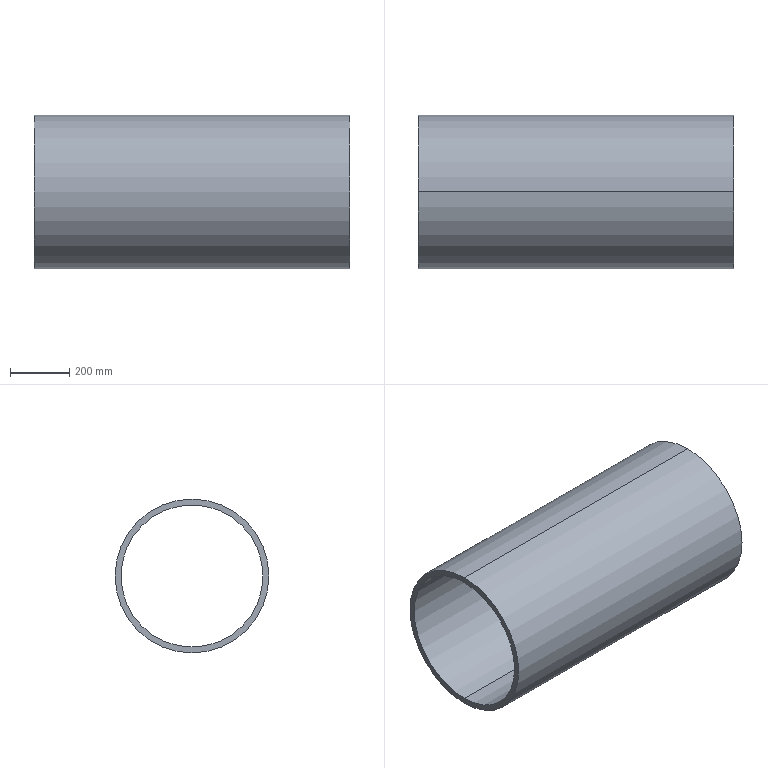Component | SolidWorks | Cev-osnovna-1 | 1 solid | 6 faces | box 1070 x 521 x 521 mm | volume 33682271 mm3 | cylinder 4 | plane 2 | commonest cylinder face diameters 481 x2 521 x2
build123d program:
from build123d import *

# Parameters (mm, degrees)
BOSS_EXTRUDE1_DEPTH      = 70
BOSS_EXTRUDE1_DEPTH_BACK = 1000
SKETCH1_R                = 260.5
SKETCH1_R_2              = 240.5


with BuildPart() as part:
    # Sketch1 → Boss-Extrude1 (new, two sides: drawn at the far end of the back side and taken through both)
    with BuildSketch(Plane.XY.offset(-7660).offset(-BOSS_EXTRUDE1_DEPTH_BACK)):
        Circle(SKETCH1_R)
        Circle(SKETCH1_R_2, mode=Mode.SUBTRACT)
    extrude(amount=BOSS_EXTRUDE1_DEPTH + BOSS_EXTRUDE1_DEPTH_BACK)


solid = part.part

# Placed as in the assembly
solid = solid.moved(Location((7660, 0, 0), (0, 90, 0)))
STEP:
#1=COLOUR_RGB('',0.7922,0.8196,0.9333);
#2=FILL_AREA_STYLE_COLOUR('',#1);
#3=FILL_AREA_STYLE('',(#2));
#4=SURFACE_STYLE_FILL_AREA(#3);
#5=SURFACE_SIDE_STYLE('',(#4));
#6=SURFACE_STYLE_USAGE(.BOTH.,#5);
#7=PRESENTATION_STYLE_ASSIGNMENT((#6));
#8=CARTESIAN_POINT('',(-39.37,0.,9.469));
#9=VERTEX_POINT('',#8);
#10=CARTESIAN_POINT('',(-39.37,0.,-9.469));
#11=VERTEX_POINT('',#10);
#12=CARTESIAN_POINT('',(-39.37,0.,-0.));
#13=DIRECTION('',(1.,0.,0.));
#14=DIRECTION('',(0.,0.,-1.));
#15=AXIS2_PLACEMENT_3D('',#12,#13,#14);
#16=CIRCLE('',#15,9.469);
#17=EDGE_CURVE('',#9,#11,#16,.T.);
#18=ORIENTED_EDGE('',*,*,#17,.F.);
#19=CARTESIAN_POINT('',(2.756,0.,9.469));
#20=VERTEX_POINT('',#19);
#21=CARTESIAN_POINT('',(-39.37,0.,9.469));
#22=DIRECTION('',(1.,0.,0.));
#23=VECTOR('',#22,39.37);
#24=LINE('',#21,#23);
#25=EDGE_CURVE('',#9,#20,#24,.T.);
#26=ORIENTED_EDGE('',*,*,#25,.T.);
#27=CARTESIAN_POINT('',(2.756,0.,-9.469));
#28=VERTEX_POINT('',#27);
#29=CARTESIAN_POINT('',(2.756,0.,0.));
#30=DIRECTION('',(1.,0.,0.));
#31=DIRECTION('',(0.,0.,-1.));
#32=AXIS2_PLACEMENT_3D('',#29,#30,#31);
#33=CIRCLE('',#32,9.469);
#34=EDGE_CURVE('',#20,#28,#33,.T.);
#35=ORIENTED_EDGE('',*,*,#34,.T.);
#36=CARTESIAN_POINT('',(-39.37,0.,-9.469));
#37=DIRECTION('',(1.,0.,0.));
#38=VECTOR('',#37,39.37);
#39=LINE('',#36,#38);
#40=EDGE_CURVE('',#11,#28,#39,.T.);
#41=ORIENTED_EDGE('',*,*,#40,.F.);
#42=EDGE_LOOP('',(#18,#26,#35,#41));
#43=FACE_OUTER_BOUND('',#42,.T.);
#44=CARTESIAN_POINT('',(-39.37,0.,-0.));
#45=DIRECTION('',(1.,0.,0.));
#46=DIRECTION('',(0.,0.,-1.));
#47=AXIS2_PLACEMENT_3D('',#44,#45,#46);
#48=CYLINDRICAL_SURFACE('',#47,9.469);
#49=ADVANCED_FACE('',(#43),#48,.F.);
#50=CARTESIAN_POINT('',(-39.37,0.,-10.256));
#51=VERTEX_POINT('',#50);
#52=CARTESIAN_POINT('',(-39.37,0.,10.256));
#53=VERTEX_POINT('',#52);
#54=CARTESIAN_POINT('',(-39.37,0.,-0.));
#55=DIRECTION('',(1.,0.,0.));
#56=DIRECTION('',(0.,0.,-1.));
#57=AXIS2_PLACEMENT_3D('',#54,#55,#56);
#58=CIRCLE('',#57,10.256);
#59=EDGE_CURVE('',#51,#53,#58,.T.);
#60=ORIENTED_EDGE('',*,*,#59,.T.);
#61=CARTESIAN_POINT('',(2.756,0.,10.256));
#62=VERTEX_POINT('',#61);
#63=CARTESIAN_POINT('',(-39.37,0.,10.256));
#64=DIRECTION('',(1.,0.,0.));
#65=VECTOR('',#64,39.37);
#66=LINE('',#63,#65);
#67=EDGE_CURVE('',#53,#62,#66,.T.);
#68=ORIENTED_EDGE('',*,*,#67,.T.);
#69=CARTESIAN_POINT('',(2.756,0.,-10.256));
#70=VERTEX_POINT('',#69);
#71=CARTESIAN_POINT('',(2.756,0.,0.));
#72=DIRECTION('',(1.,0.,0.));
#73=DIRECTION('',(0.,0.,-1.));
#74=AXIS2_PLACEMENT_3D('',#71,#72,#73);
#75=CIRCLE('',#74,10.256);
#76=EDGE_CURVE('',#70,#62,#75,.T.);
#77=ORIENTED_EDGE('',*,*,#76,.F.);
#78=CARTESIAN_POINT('',(-39.37,0.,-10.256));
#79=DIRECTION('',(1.,0.,0.));
#80=VECTOR('',#79,39.37);
#81=LINE('',#78,#80);
#82=EDGE_CURVE('',#51,#70,#81,.T.);
#83=ORIENTED_EDGE('',*,*,#82,.F.);
#84=EDGE_LOOP('',(#60,#68,#77,#83));
#85=FACE_OUTER_BOUND('',#84,.T.);
#86=CARTESIAN_POINT('',(-39.37,0.,-0.));
#87=DIRECTION('',(1.,0.,0.));
#88=DIRECTION('',(0.,0.,-1.));
#89=AXIS2_PLACEMENT_3D('',#86,#87,#88);
#90=CYLINDRICAL_SURFACE('',#89,10.256);
#91=ADVANCED_FACE('',(#85),#90,.T.);
#92=ORIENTED_EDGE('',*,*,#67,.F.);
#93=CARTESIAN_POINT('',(-39.37,0.,-0.));
#94=DIRECTION('',(1.,0.,0.));
#95=DIRECTION('',(0.,0.,-1.));
#96=AXIS2_PLACEMENT_3D('',#93,#94,#95);
#97=CIRCLE('',#96,10.256);
#98=EDGE_CURVE('',#53,#51,#97,.T.);
#99=ORIENTED_EDGE('',*,*,#98,.T.);
#100=ORIENTED_EDGE('',*,*,#82,.T.);
#101=CARTESIAN_POINT('',(2.756,0.,0.));
#102=DIRECTION('',(1.,0.,0.));
#103=DIRECTION('',(0.,0.,-1.));
#104=AXIS2_PLACEMENT_3D('',#101,#102,#103);
#105=CIRCLE('',#104,10.256);
#106=EDGE_CURVE('',#62,#70,#105,.T.);
#107=ORIENTED_EDGE('',*,*,#106,.F.);
#108=EDGE_LOOP('',(#92,#99,#100,#107));
#109=FACE_OUTER_BOUND('',#108,.T.);
#110=CARTESIAN_POINT('',(-39.37,0.,-0.));
#111=DIRECTION('',(1.,0.,0.));
#112=DIRECTION('',(0.,0.,-1.));
#113=AXIS2_PLACEMENT_3D('',#110,#111,#112);
#114=CYLINDRICAL_SURFACE('',#113,10.256);
#115=ADVANCED_FACE('',(#109),#114,.T.);
#116=CARTESIAN_POINT('',(-39.37,0.,-0.));
#117=DIRECTION('',(1.,0.,0.));
#118=DIRECTION('',(0.,0.,-1.));
#119=AXIS2_PLACEMENT_3D('',#116,#117,#118);
#120=CIRCLE('',#119,9.469);
#121=EDGE_CURVE('',#11,#9,#120,.T.);
#122=ORIENTED_EDGE('',*,*,#121,.T.);
#123=ORIENTED_EDGE('',*,*,#17,.T.);
#124=EDGE_LOOP('',(#122,#123));
#125=FACE_BOUND('',#124,.T.);
#126=ORIENTED_EDGE('',*,*,#59,.F.);
#127=ORIENTED_EDGE('',*,*,#98,.F.);
#128=EDGE_LOOP('',(#126,#127));
#129=FACE_OUTER_BOUND('',#128,.T.);
#130=CARTESIAN_POINT('',(-39.37,0.,-0.));
#131=DIRECTION('',(1.,0.,0.));
#132=DIRECTION('',(0.,0.,-1.));
#133=AXIS2_PLACEMENT_3D('',#130,#131,#132);
#134=PLANE('',#133);
#135=ADVANCED_FACE('',(#125,#129),#134,.F.);
#136=ORIENTED_EDGE('',*,*,#25,.F.);
#137=ORIENTED_EDGE('',*,*,#121,.F.);
#138=ORIENTED_EDGE('',*,*,#40,.T.);
#139=CARTESIAN_POINT('',(2.756,0.,0.));
#140=DIRECTION('',(1.,0.,0.));
#141=DIRECTION('',(0.,0.,-1.));
#142=AXIS2_PLACEMENT_3D('',#139,#140,#141);
#143=CIRCLE('',#142,9.469);
#144=EDGE_CURVE('',#28,#20,#143,.T.);
#145=ORIENTED_EDGE('',*,*,#144,.T.);
#146=EDGE_LOOP('',(#136,#137,#138,#145));
#147=FACE_OUTER_BOUND('',#146,.T.);
#148=CARTESIAN_POINT('',(-39.37,0.,-0.));
#149=DIRECTION('',(1.,0.,0.));
#150=DIRECTION('',(0.,0.,-1.));
#151=AXIS2_PLACEMENT_3D('',#148,#149,#150);
#152=CYLINDRICAL_SURFACE('',#151,9.469);
#153=ADVANCED_FACE('',(#147),#152,.F.);
#154=ORIENTED_EDGE('',*,*,#76,.T.);
#155=ORIENTED_EDGE('',*,*,#106,.T.);
#156=EDGE_LOOP('',(#154,#155));
#157=FACE_OUTER_BOUND('',#156,.T.);
#158=ORIENTED_EDGE('',*,*,#144,.F.);
#159=ORIENTED_EDGE('',*,*,#34,.F.);
#160=EDGE_LOOP('',(#158,#159));
#161=FACE_BOUND('',#160,.T.);
#162=CARTESIAN_POINT('',(2.756,0.,0.));
#163=DIRECTION('',(1.,0.,0.));
#164=DIRECTION('',(0.,0.,-1.));
#165=AXIS2_PLACEMENT_3D('',#162,#163,#164);
#166=PLANE('',#165);
#167=ADVANCED_FACE('',(#157,#161),#166,.T.);
#168=CLOSED_SHELL('',(#49,#91,#115,#135,#153,#167));
#169=MANIFOLD_SOLID_BREP('',#168);
#170=STYLED_ITEM('',(#7),#169);
#171=(LENGTH_UNIT()NAMED_UNIT(*)SI_UNIT($,.METRE.));
#172=LENGTH_MEASURE_WITH_UNIT(LENGTH_MEASURE(0.0254),#171);
#173=DIMENSIONAL_EXPONENTS(1.,0.,0.,0.,0.,0.,0.);
#174=(CONVERSION_BASED_UNIT('',#172)LENGTH_UNIT()NAMED_UNIT(#173));
#175=UNCERTAINTY_MEASURE_WITH_UNIT(LENGTH_MEASURE(0.00001),#174,'','');
#176=(NAMED_UNIT(*)PLANE_ANGLE_UNIT()SI_UNIT($,.RADIAN.));
#177=(NAMED_UNIT(*)SI_UNIT($,.STERADIAN.)SOLID_ANGLE_UNIT());
#178=(GEOMETRIC_REPRESENTATION_CONTEXT(3)GLOBAL_UNCERTAINTY_ASSIGNED_CONTEXT((#175))GLOBAL_UNIT_ASSIGNED_CONTEXT((#174,#176,#177))REPRESENTATION_CONTEXT('',''));
#179=MECHANICAL_DESIGN_GEOMETRIC_PRESENTATION_REPRESENTATION('',(#170),#178);
#180=CARTESIAN_POINT('',(0.,0.,0.));
#181=DIRECTION('',(0.,0.,1.));
#182=DIRECTION('',(1.,0.,0.));
#183=AXIS2_PLACEMENT_3D('',#180,#181,#182);
#184=(LENGTH_UNIT()NAMED_UNIT(*)SI_UNIT($,.METRE.));
#185=LENGTH_MEASURE_WITH_UNIT(LENGTH_MEASURE(0.0254),#184);
#186=DIMENSIONAL_EXPONENTS(1.,0.,0.,0.,0.,0.,0.);
#187=(CONVERSION_BASED_UNIT('',#185)LENGTH_UNIT()NAMED_UNIT(#186));
#188=UNCERTAINTY_MEASURE_WITH_UNIT(LENGTH_MEASURE(0.00001),#187,'','');
#189=(NAMED_UNIT(*)PLANE_ANGLE_UNIT()SI_UNIT($,.RADIAN.));
#190=(NAMED_UNIT(*)SI_UNIT($,.STERADIAN.)SOLID_ANGLE_UNIT());
#191=(GEOMETRIC_REPRESENTATION_CONTEXT(3)GLOBAL_UNCERTAINTY_ASSIGNED_CONTEXT((#188))GLOBAL_UNIT_ASSIGNED_CONTEXT((#187,#189,#190))REPRESENTATION_CONTEXT('',''));
#192=ADVANCED_BREP_SHAPE_REPRESENTATION('',(#169,#183),#191);
#193=PRESENTATION_LAYER_ASSIGNMENT('','',(#170));